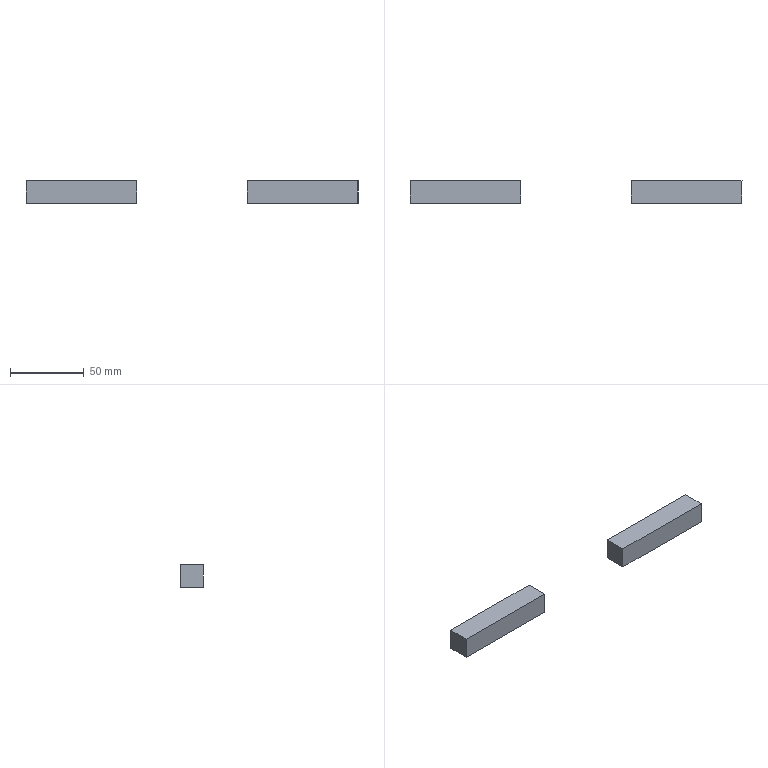Component | SolidWorks | Press-inFixture1-1 | 2 solids | 28 faces | box 225 x 15 x 15 mm | volume 33345 mm3 | plane 12 | cylinder 8 | cone 8 | commonest cylinder face diameters 3.3 x8
build123d program:
from build123d import *

# Parameters (mm, degrees)
SKETCH1_W             = 75
SKETCH1_H             = 15
BOSS_EXTRUDE1_DEPTH   = 15
M4_TAPPED_HOLE2_D     = 3.3
M4_TAPPED_HOLE2_DEPTH = 11.5
M4_TAPPED_HOLE2_TIP   = 0.9914


with BuildPart() as part:
    # Sketch1 → Boss-Extrude1 (new body)
    with BuildSketch(Plane(origin=(0, 0, 0), x_dir=(1, 0, 0), z_dir=(0, 1, 0))):
        Rectangle(SKETCH1_W, SKETCH1_H)
    extrude(amount=BOSS_EXTRUDE1_DEPTH)

    # M4 Tapped Hole2
    with Locations(Plane(origin=(0, 0, 0), x_dir=(-1, 0, 0), z_dir=(0, -1, 0))):
        with Locations((-22.5, 1.5), (22.5, 1.5)):
            Hole(M4_TAPPED_HOLE2_D / 2, depth=M4_TAPPED_HOLE2_DEPTH)
            with Locations((0, 0, -(M4_TAPPED_HOLE2_DEPTH + M4_TAPPED_HOLE2_TIP / 2))):  # 118° drill point
                Cone(0, M4_TAPPED_HOLE2_D / 2, M4_TAPPED_HOLE2_TIP, mode=Mode.SUBTRACT)


with BuildPart() as body_2:
    # Mirror2: mirrored copy
    add(part.part.mirror(Plane.ZY.offset(-75)))


solid = Compound([part.part, body_2.part])

# Placed as in the assembly
solid = solid.moved(Location((-45, -65.5, 208.602), (180, 0, 0)))
STEP:
#1=COLOUR_RGB('',0.7922,0.8196,0.9333);
#2=FILL_AREA_STYLE_COLOUR('',#1);
#3=FILL_AREA_STYLE('',(#2));
#4=SURFACE_STYLE_FILL_AREA(#3);
#5=SURFACE_SIDE_STYLE('',(#4));
#6=SURFACE_STYLE_USAGE(.BOTH.,#5);
#7=PRESENTATION_STYLE_ASSIGNMENT((#6));
#8=CARTESIAN_POINT('',(-0.8858,-3.031,8.207));
#9=VERTEX_POINT('',#8);
#10=CARTESIAN_POINT('',(-0.8858,-3.031,8.337));
#11=VERTEX_POINT('',#10);
#12=CARTESIAN_POINT('',(-0.8858,-3.031,8.272));
#13=DIRECTION('',(-0.,1.,0.));
#14=DIRECTION('',(0.,0.,1.));
#15=AXIS2_PLACEMENT_3D('',#12,#13,#14);
#16=CIRCLE('',#15,0.06496);
#17=EDGE_CURVE('',#9,#11,#16,.T.);
#18=ORIENTED_EDGE('',*,*,#17,.F.);
#19=CARTESIAN_POINT('',(-0.8858,-2.579,8.207));
#20=VERTEX_POINT('',#19);
#21=CARTESIAN_POINT('',(-0.8858,-2.579,8.207));
#22=DIRECTION('',(-0.,1.,0.));
#23=VECTOR('',#22,39.37);
#24=LINE('',#21,#23);
#25=EDGE_CURVE('',#9,#20,#24,.T.);
#26=ORIENTED_EDGE('',*,*,#25,.T.);
#27=CARTESIAN_POINT('',(-0.8858,-2.579,8.337));
#28=VERTEX_POINT('',#27);
#29=CARTESIAN_POINT('',(-0.8858,-2.579,8.272));
#30=DIRECTION('',(-0.,1.,0.));
#31=DIRECTION('',(0.,0.,1.));
#32=AXIS2_PLACEMENT_3D('',#29,#30,#31);
#33=CIRCLE('',#32,0.06496);
#34=EDGE_CURVE('',#20,#28,#33,.T.);
#35=ORIENTED_EDGE('',*,*,#34,.T.);
#36=CARTESIAN_POINT('',(-0.8858,-2.579,8.337));
#37=DIRECTION('',(-0.,1.,0.));
#38=VECTOR('',#37,39.37);
#39=LINE('',#36,#38);
#40=EDGE_CURVE('',#11,#28,#39,.T.);
#41=ORIENTED_EDGE('',*,*,#40,.F.);
#42=EDGE_LOOP('',(#18,#26,#35,#41));
#43=FACE_OUTER_BOUND('',#42,.T.);
#44=CARTESIAN_POINT('',(-0.8858,-2.579,8.272));
#45=DIRECTION('',(-0.,1.,0.));
#46=DIRECTION('',(0.,0.,1.));
#47=AXIS2_PLACEMENT_3D('',#44,#45,#46);
#48=CYLINDRICAL_SURFACE('',#47,0.06496);
#49=ADVANCED_FACE('',(#43),#48,.F.);
#50=CARTESIAN_POINT('',(-0.8858,-3.071,8.272));
#51=VERTEX_POINT('',#50);
#52=CARTESIAN_POINT('',(-0.8858,-3.031,8.337));
#53=DIRECTION('',(-0.,0.515,0.8572));
#54=VECTOR('',#53,39.37);
#55=LINE('',#52,#54);
#56=EDGE_CURVE('',#51,#11,#55,.T.);
#57=ORIENTED_EDGE('',*,*,#56,.F.);
#58=CARTESIAN_POINT('',(-0.8858,-3.031,8.207));
#59=DIRECTION('',(-0.,0.515,-0.8572));
#60=VECTOR('',#59,39.37);
#61=LINE('',#58,#60);
#62=EDGE_CURVE('',#51,#9,#61,.T.);
#63=ORIENTED_EDGE('',*,*,#62,.T.);
#64=ORIENTED_EDGE('',*,*,#17,.T.);
#65=EDGE_LOOP('',(#57,#63,#64));
#66=FACE_OUTER_BOUND('',#65,.T.);
#67=CARTESIAN_POINT('',(-0.8858,-3.031,8.272));
#68=DIRECTION('',(-0.,1.,0.));
#69=DIRECTION('',(0.,0.,1.));
#70=AXIS2_PLACEMENT_3D('',#67,#68,#69);
#71=CONICAL_SURFACE('',#70,0.06496,1.03);
#72=ADVANCED_FACE('',(#66),#71,.F.);
#73=CARTESIAN_POINT('',(-2.657,-3.031,8.207));
#74=VERTEX_POINT('',#73);
#75=CARTESIAN_POINT('',(-2.657,-3.031,8.337));
#76=VERTEX_POINT('',#75);
#77=CARTESIAN_POINT('',(-2.657,-3.031,8.272));
#78=DIRECTION('',(-0.,1.,0.));
#79=DIRECTION('',(0.,0.,1.));
#80=AXIS2_PLACEMENT_3D('',#77,#78,#79);
#81=CIRCLE('',#80,0.06496);
#82=EDGE_CURVE('',#74,#76,#81,.T.);
#83=ORIENTED_EDGE('',*,*,#82,.F.);
#84=CARTESIAN_POINT('',(-2.657,-2.579,8.207));
#85=VERTEX_POINT('',#84);
#86=CARTESIAN_POINT('',(-2.657,-2.579,8.207));
#87=DIRECTION('',(-0.,1.,0.));
#88=VECTOR('',#87,39.37);
#89=LINE('',#86,#88);
#90=EDGE_CURVE('',#74,#85,#89,.T.);
#91=ORIENTED_EDGE('',*,*,#90,.T.);
#92=CARTESIAN_POINT('',(-2.657,-2.579,8.337));
#93=VERTEX_POINT('',#92);
#94=CARTESIAN_POINT('',(-2.657,-2.579,8.272));
#95=DIRECTION('',(-0.,1.,0.));
#96=DIRECTION('',(0.,0.,1.));
#97=AXIS2_PLACEMENT_3D('',#94,#95,#96);
#98=CIRCLE('',#97,0.06496);
#99=EDGE_CURVE('',#85,#93,#98,.T.);
#100=ORIENTED_EDGE('',*,*,#99,.T.);
#101=CARTESIAN_POINT('',(-2.657,-2.579,8.337));
#102=DIRECTION('',(-0.,1.,0.));
#103=VECTOR('',#102,39.37);
#104=LINE('',#101,#103);
#105=EDGE_CURVE('',#76,#93,#104,.T.);
#106=ORIENTED_EDGE('',*,*,#105,.F.);
#107=EDGE_LOOP('',(#83,#91,#100,#106));
#108=FACE_OUTER_BOUND('',#107,.T.);
#109=CARTESIAN_POINT('',(-2.657,-2.579,8.272));
#110=DIRECTION('',(-0.,1.,0.));
#111=DIRECTION('',(0.,0.,1.));
#112=AXIS2_PLACEMENT_3D('',#109,#110,#111);
#113=CYLINDRICAL_SURFACE('',#112,0.06496);
#114=ADVANCED_FACE('',(#108),#113,.F.);
#115=CARTESIAN_POINT('',(-2.657,-3.071,8.272));
#116=VERTEX_POINT('',#115);
#117=CARTESIAN_POINT('',(-2.657,-3.031,8.337));
#118=DIRECTION('',(-0.,0.515,0.8572));
#119=VECTOR('',#118,39.37);
#120=LINE('',#117,#119);
#121=EDGE_CURVE('',#116,#76,#120,.T.);
#122=ORIENTED_EDGE('',*,*,#121,.F.);
#123=CARTESIAN_POINT('',(-2.657,-3.031,8.207));
#124=DIRECTION('',(-0.,0.515,-0.8572));
#125=VECTOR('',#124,39.37);
#126=LINE('',#123,#125);
#127=EDGE_CURVE('',#116,#74,#126,.T.);
#128=ORIENTED_EDGE('',*,*,#127,.T.);
#129=ORIENTED_EDGE('',*,*,#82,.T.);
#130=EDGE_LOOP('',(#122,#128,#129));
#131=FACE_OUTER_BOUND('',#130,.T.);
#132=CARTESIAN_POINT('',(-2.657,-3.031,8.272));
#133=DIRECTION('',(-0.,1.,0.));
#134=DIRECTION('',(0.,0.,1.));
#135=AXIS2_PLACEMENT_3D('',#132,#133,#134);
#136=CONICAL_SURFACE('',#135,0.06496,1.03);
#137=ADVANCED_FACE('',(#131),#136,.F.);
#138=CARTESIAN_POINT('',(-3.248,-2.579,8.508));
#139=VERTEX_POINT('',#138);
#140=CARTESIAN_POINT('',(-3.248,-2.579,7.917));
#141=VERTEX_POINT('',#140);
#142=CARTESIAN_POINT('',(-3.248,-2.579,7.917));
#143=DIRECTION('',(-0.,0.,-1.));
#144=VECTOR('',#143,39.37);
#145=LINE('',#142,#144);
#146=EDGE_CURVE('',#139,#141,#145,.T.);
#147=ORIENTED_EDGE('',*,*,#146,.T.);
#148=CARTESIAN_POINT('',(-3.248,-3.169,7.917));
#149=VERTEX_POINT('',#148);
#150=CARTESIAN_POINT('',(-3.248,-3.169,7.917));
#151=DIRECTION('',(-0.,1.,0.));
#152=VECTOR('',#151,39.37);
#153=LINE('',#150,#152);
#154=EDGE_CURVE('',#149,#141,#153,.T.);
#155=ORIENTED_EDGE('',*,*,#154,.F.);
#156=CARTESIAN_POINT('',(-3.248,-3.169,8.508));
#157=VERTEX_POINT('',#156);
#158=CARTESIAN_POINT('',(-3.248,-3.169,7.917));
#159=DIRECTION('',(-0.,0.,-1.));
#160=VECTOR('',#159,39.37);
#161=LINE('',#158,#160);
#162=EDGE_CURVE('',#157,#149,#161,.T.);
#163=ORIENTED_EDGE('',*,*,#162,.F.);
#164=CARTESIAN_POINT('',(-3.248,-3.169,8.508));
#165=DIRECTION('',(-0.,1.,0.));
#166=VECTOR('',#165,39.37);
#167=LINE('',#164,#166);
#168=EDGE_CURVE('',#157,#139,#167,.T.);
#169=ORIENTED_EDGE('',*,*,#168,.T.);
#170=EDGE_LOOP('',(#147,#155,#163,#169));
#171=FACE_OUTER_BOUND('',#170,.T.);
#172=CARTESIAN_POINT('',(-3.248,-3.169,7.917));
#173=DIRECTION('',(1.,0.,-0.));
#174=DIRECTION('',(0.,-0.,1.));
#175=AXIS2_PLACEMENT_3D('',#172,#173,#174);
#176=PLANE('',#175);
#177=ADVANCED_FACE('',(#171),#176,.F.);
#178=CARTESIAN_POINT('',(-0.2953,-2.579,7.917));
#179=VERTEX_POINT('',#178);
#180=CARTESIAN_POINT('',(-0.2953,-2.579,7.917));
#181=DIRECTION('',(1.,0.,0.));
#182=VECTOR('',#181,39.37);
#183=LINE('',#180,#182);
#184=EDGE_CURVE('',#141,#179,#183,.T.);
#185=ORIENTED_EDGE('',*,*,#184,.T.);
#186=CARTESIAN_POINT('',(-0.2953,-3.169,7.917));
#187=VERTEX_POINT('',#186);
#188=CARTESIAN_POINT('',(-0.2953,-3.169,7.917));
#189=DIRECTION('',(-0.,1.,0.));
#190=VECTOR('',#189,39.37);
#191=LINE('',#188,#190);
#192=EDGE_CURVE('',#187,#179,#191,.T.);
#193=ORIENTED_EDGE('',*,*,#192,.F.);
#194=CARTESIAN_POINT('',(-0.2953,-3.169,7.917));
#195=DIRECTION('',(1.,0.,0.));
#196=VECTOR('',#195,39.37);
#197=LINE('',#194,#196);
#198=EDGE_CURVE('',#149,#187,#197,.T.);
#199=ORIENTED_EDGE('',*,*,#198,.F.);
#200=ORIENTED_EDGE('',*,*,#154,.T.);
#201=EDGE_LOOP('',(#185,#193,#199,#200));
#202=FACE_OUTER_BOUND('',#201,.T.);
#203=CARTESIAN_POINT('',(-0.2953,-3.169,7.917));
#204=DIRECTION('',(-0.,-0.,1.));
#205=DIRECTION('',(-1.,-0.,-0.));
#206=AXIS2_PLACEMENT_3D('',#203,#204,#205);
#207=PLANE('',#206);
#208=ADVANCED_FACE('',(#202),#207,.F.);
#209=CARTESIAN_POINT('',(-0.2953,-2.579,8.508));
#210=VERTEX_POINT('',#209);
#211=CARTESIAN_POINT('',(-0.2953,-2.579,7.917));
#212=DIRECTION('',(0.,-0.,1.));
#213=VECTOR('',#212,39.37);
#214=LINE('',#211,#213);
#215=EDGE_CURVE('',#179,#210,#214,.T.);
#216=ORIENTED_EDGE('',*,*,#215,.T.);
#217=CARTESIAN_POINT('',(-0.2953,-3.169,8.508));
#218=VERTEX_POINT('',#217);
#219=CARTESIAN_POINT('',(-0.2953,-3.169,8.508));
#220=DIRECTION('',(-0.,1.,0.));
#221=VECTOR('',#220,39.37);
#222=LINE('',#219,#221);
#223=EDGE_CURVE('',#218,#210,#222,.T.);
#224=ORIENTED_EDGE('',*,*,#223,.F.);
#225=CARTESIAN_POINT('',(-0.2953,-3.169,7.917));
#226=DIRECTION('',(0.,-0.,1.));
#227=VECTOR('',#226,39.37);
#228=LINE('',#225,#227);
#229=EDGE_CURVE('',#187,#218,#228,.T.);
#230=ORIENTED_EDGE('',*,*,#229,.F.);
#231=ORIENTED_EDGE('',*,*,#192,.T.);
#232=EDGE_LOOP('',(#216,#224,#230,#231));
#233=FACE_OUTER_BOUND('',#232,.T.);
#234=CARTESIAN_POINT('',(-0.2953,-3.169,7.917));
#235=DIRECTION('',(-1.,-0.,0.));
#236=DIRECTION('',(-0.,0.,-1.));
#237=AXIS2_PLACEMENT_3D('',#234,#235,#236);
#238=PLANE('',#237);
#239=ADVANCED_FACE('',(#233),#238,.F.);
#240=CARTESIAN_POINT('',(-0.2953,-2.579,8.508));
#241=DIRECTION('',(-1.,-0.,-0.));
#242=VECTOR('',#241,39.37);
#243=LINE('',#240,#242);
#244=EDGE_CURVE('',#210,#139,#243,.T.);
#245=ORIENTED_EDGE('',*,*,#244,.T.);
#246=ORIENTED_EDGE('',*,*,#168,.F.);
#247=CARTESIAN_POINT('',(-0.2953,-3.169,8.508));
#248=DIRECTION('',(-1.,-0.,-0.));
#249=VECTOR('',#248,39.37);
#250=LINE('',#247,#249);
#251=EDGE_CURVE('',#218,#157,#250,.T.);
#252=ORIENTED_EDGE('',*,*,#251,.F.);
#253=ORIENTED_EDGE('',*,*,#223,.T.);
#254=EDGE_LOOP('',(#245,#246,#252,#253));
#255=FACE_OUTER_BOUND('',#254,.T.);
#256=CARTESIAN_POINT('',(-0.2953,-3.169,8.508));
#257=DIRECTION('',(0.,0.,-1.));
#258=DIRECTION('',(1.,0.,0.));
#259=AXIS2_PLACEMENT_3D('',#256,#257,#258);
#260=PLANE('',#259);
#261=ADVANCED_FACE('',(#255),#260,.F.);
#262=ORIENTED_EDGE('',*,*,#162,.T.);
#263=ORIENTED_EDGE('',*,*,#198,.T.);
#264=ORIENTED_EDGE('',*,*,#229,.T.);
#265=ORIENTED_EDGE('',*,*,#251,.T.);
#266=EDGE_LOOP('',(#262,#263,#264,#265));
#267=FACE_OUTER_BOUND('',#266,.T.);
#268=CARTESIAN_POINT('',(-1.772,-3.169,8.213));
#269=DIRECTION('',(0.,-1.,-0.));
#270=DIRECTION('',(-0.,0.,-1.));
#271=AXIS2_PLACEMENT_3D('',#268,#269,#270);
#272=PLANE('',#271);
#273=ADVANCED_FACE('',(#267),#272,.T.);
#274=CARTESIAN_POINT('',(-0.8858,-2.579,8.272));
#275=DIRECTION('',(-0.,1.,0.));
#276=DIRECTION('',(0.,0.,1.));
#277=AXIS2_PLACEMENT_3D('',#274,#275,#276);
#278=CIRCLE('',#277,0.06496);
#279=EDGE_CURVE('',#28,#20,#278,.T.);
#280=ORIENTED_EDGE('',*,*,#279,.F.);
#281=ORIENTED_EDGE('',*,*,#34,.F.);
#282=EDGE_LOOP('',(#280,#281));
#283=FACE_BOUND('',#282,.T.);
#284=CARTESIAN_POINT('',(-2.657,-2.579,8.272));
#285=DIRECTION('',(-0.,1.,0.));
#286=DIRECTION('',(0.,0.,1.));
#287=AXIS2_PLACEMENT_3D('',#284,#285,#286);
#288=CIRCLE('',#287,0.06496);
#289=EDGE_CURVE('',#93,#85,#288,.T.);
#290=ORIENTED_EDGE('',*,*,#289,.F.);
#291=ORIENTED_EDGE('',*,*,#99,.F.);
#292=EDGE_LOOP('',(#290,#291));
#293=FACE_BOUND('',#292,.T.);
#294=ORIENTED_EDGE('',*,*,#146,.F.);
#295=ORIENTED_EDGE('',*,*,#244,.F.);
#296=ORIENTED_EDGE('',*,*,#215,.F.);
#297=ORIENTED_EDGE('',*,*,#184,.F.);
#298=EDGE_LOOP('',(#294,#295,#296,#297));
#299=FACE_OUTER_BOUND('',#298,.T.);
#300=CARTESIAN_POINT('',(-1.772,-2.579,8.213));
#301=DIRECTION('',(0.,-1.,-0.));
#302=DIRECTION('',(-0.,0.,-1.));
#303=AXIS2_PLACEMENT_3D('',#300,#301,#302);
#304=PLANE('',#303);
#305=ADVANCED_FACE('',(#283,#293,#299),#304,.F.);
#306=ORIENTED_EDGE('',*,*,#127,.F.);
#307=ORIENTED_EDGE('',*,*,#121,.T.);
#308=CARTESIAN_POINT('',(-2.657,-3.031,8.272));
#309=DIRECTION('',(-0.,1.,0.));
#310=DIRECTION('',(0.,0.,1.));
#311=AXIS2_PLACEMENT_3D('',#308,#309,#310);
#312=CIRCLE('',#311,0.06496);
#313=EDGE_CURVE('',#76,#74,#312,.T.);
#314=ORIENTED_EDGE('',*,*,#313,.T.);
#315=EDGE_LOOP('',(#306,#307,#314));
#316=FACE_OUTER_BOUND('',#315,.T.);
#317=CARTESIAN_POINT('',(-2.657,-3.031,8.272));
#318=DIRECTION('',(-0.,1.,0.));
#319=DIRECTION('',(0.,0.,1.));
#320=AXIS2_PLACEMENT_3D('',#317,#318,#319);
#321=CONICAL_SURFACE('',#320,0.06496,1.03);
#322=ADVANCED_FACE('',(#316),#321,.F.);
#323=ORIENTED_EDGE('',*,*,#90,.F.);
#324=ORIENTED_EDGE('',*,*,#313,.F.);
#325=ORIENTED_EDGE('',*,*,#105,.T.);
#326=ORIENTED_EDGE('',*,*,#289,.T.);
#327=EDGE_LOOP('',(#323,#324,#325,#326));
#328=FACE_OUTER_BOUND('',#327,.T.);
#329=CARTESIAN_POINT('',(-2.657,-2.579,8.272));
#330=DIRECTION('',(-0.,1.,0.));
#331=DIRECTION('',(0.,0.,1.));
#332=AXIS2_PLACEMENT_3D('',#329,#330,#331);
#333=CYLINDRICAL_SURFACE('',#332,0.06496);
#334=ADVANCED_FACE('',(#328),#333,.F.);
#335=ORIENTED_EDGE('',*,*,#62,.F.);
#336=ORIENTED_EDGE('',*,*,#56,.T.);
#337=CARTESIAN_POINT('',(-0.8858,-3.031,8.272));
#338=DIRECTION('',(-0.,1.,0.));
#339=DIRECTION('',(0.,0.,1.));
#340=AXIS2_PLACEMENT_3D('',#337,#338,#339);
#341=CIRCLE('',#340,0.06496);
#342=EDGE_CURVE('',#11,#9,#341,.T.);
#343=ORIENTED_EDGE('',*,*,#342,.T.);
#344=EDGE_LOOP('',(#335,#336,#343));
#345=FACE_OUTER_BOUND('',#344,.T.);
#346=CARTESIAN_POINT('',(-0.8858,-3.031,8.272));
#347=DIRECTION('',(-0.,1.,0.));
#348=DIRECTION('',(0.,0.,1.));
#349=AXIS2_PLACEMENT_3D('',#346,#347,#348);
#350=CONICAL_SURFACE('',#349,0.06496,1.03);
#351=ADVANCED_FACE('',(#345),#350,.F.);
#352=ORIENTED_EDGE('',*,*,#25,.F.);
#353=ORIENTED_EDGE('',*,*,#342,.F.);
#354=ORIENTED_EDGE('',*,*,#40,.T.);
#355=ORIENTED_EDGE('',*,*,#279,.T.);
#356=EDGE_LOOP('',(#352,#353,#354,#355));
#357=FACE_OUTER_BOUND('',#356,.T.);
#358=CARTESIAN_POINT('',(-0.8858,-2.579,8.272));
#359=DIRECTION('',(-0.,1.,0.));
#360=DIRECTION('',(0.,0.,1.));
#361=AXIS2_PLACEMENT_3D('',#358,#359,#360);
#362=CYLINDRICAL_SURFACE('',#361,0.06496);
#363=ADVANCED_FACE('',(#357),#362,.F.);
#364=CLOSED_SHELL('',(#49,#72,#114,#137,#177,#208,#239,#261,#273,#305,#322,#334,#351,#363));
#365=MANIFOLD_SOLID_BREP('',#364);
#366=STYLED_ITEM('',(#7),#365);
#367=PRESENTATION_LAYER_ASSIGNMENT('','',(#366));
#368=(LENGTH_UNIT()NAMED_UNIT(*)SI_UNIT($,.METRE.));
#369=LENGTH_MEASURE_WITH_UNIT(LENGTH_MEASURE(0.0254),#368);
#370=DIMENSIONAL_EXPONENTS(1.,0.,0.,0.,0.,0.,0.);
#371=(CONVERSION_BASED_UNIT('',#369)LENGTH_UNIT()NAMED_UNIT(#370));
#372=UNCERTAINTY_MEASURE_WITH_UNIT(LENGTH_MEASURE(0.00001),#371,'','');
#373=(NAMED_UNIT(*)PLANE_ANGLE_UNIT()SI_UNIT($,.RADIAN.));
#374=(NAMED_UNIT(*)SI_UNIT($,.STERADIAN.)SOLID_ANGLE_UNIT());
#375=(GEOMETRIC_REPRESENTATION_CONTEXT(3)GLOBAL_UNCERTAINTY_ASSIGNED_CONTEXT((#372))GLOBAL_UNIT_ASSIGNED_CONTEXT((#371,#373,#374))REPRESENTATION_CONTEXT('',''));
#376=MECHANICAL_DESIGN_GEOMETRIC_PRESENTATION_REPRESENTATION('',(#366),#375);
#377=CARTESIAN_POINT('',(3.248,-3.031,8.337));
#378=VERTEX_POINT('',#377);
#379=CARTESIAN_POINT('',(3.248,-3.031,8.207));
#380=VERTEX_POINT('',#379);
#381=CARTESIAN_POINT('',(3.248,-3.031,8.272));
#382=DIRECTION('',(-0.,-1.,-0.));
#383=DIRECTION('',(0.,0.,1.));
#384=AXIS2_PLACEMENT_3D('',#381,#382,#383);
#385=CIRCLE('',#384,0.06496);
#386=EDGE_CURVE('',#378,#380,#385,.T.);
#387=ORIENTED_EDGE('',*,*,#386,.T.);
#388=CARTESIAN_POINT('',(3.248,-2.579,8.207));
#389=VERTEX_POINT('',#388);
#390=CARTESIAN_POINT('',(3.248,-2.579,8.207));
#391=DIRECTION('',(0.,1.,0.));
#392=VECTOR('',#391,39.37);
#393=LINE('',#390,#392);
#394=EDGE_CURVE('',#380,#389,#393,.T.);
#395=ORIENTED_EDGE('',*,*,#394,.T.);
#396=CARTESIAN_POINT('',(3.248,-2.579,8.337));
#397=VERTEX_POINT('',#396);
#398=CARTESIAN_POINT('',(3.248,-2.579,8.272));
#399=DIRECTION('',(-0.,-1.,-0.));
#400=DIRECTION('',(0.,0.,1.));
#401=AXIS2_PLACEMENT_3D('',#398,#399,#400);
#402=CIRCLE('',#401,0.06496);
#403=EDGE_CURVE('',#397,#389,#402,.T.);
#404=ORIENTED_EDGE('',*,*,#403,.F.);
#405=CARTESIAN_POINT('',(3.248,-2.579,8.337));
#406=DIRECTION('',(0.,1.,0.));
#407=VECTOR('',#406,39.37);
#408=LINE('',#405,#407);
#409=EDGE_CURVE('',#378,#397,#408,.T.);
#410=ORIENTED_EDGE('',*,*,#409,.F.);
#411=EDGE_LOOP('',(#387,#395,#404,#410));
#412=FACE_OUTER_BOUND('',#411,.T.);
#413=CARTESIAN_POINT('',(3.248,-2.579,8.272));
#414=DIRECTION('',(0.,1.,0.));
#415=DIRECTION('',(0.,0.,1.));
#416=AXIS2_PLACEMENT_3D('',#413,#414,#415);
#417=CYLINDRICAL_SURFACE('',#416,0.06496);
#418=ADVANCED_FACE('',(#412),#417,.F.);
#419=CARTESIAN_POINT('',(3.248,-3.071,8.272));
#420=VERTEX_POINT('',#419);
#421=CARTESIAN_POINT('',(3.248,-3.031,8.337));
#422=DIRECTION('',(0.,0.515,0.8572));
#423=VECTOR('',#422,39.37);
#424=LINE('',#421,#423);
#425=EDGE_CURVE('',#420,#378,#424,.T.);
#426=ORIENTED_EDGE('',*,*,#425,.F.);
#427=CARTESIAN_POINT('',(3.248,-3.031,8.207));
#428=DIRECTION('',(0.,0.515,-0.8572));
#429=VECTOR('',#428,39.37);
#430=LINE('',#427,#429);
#431=EDGE_CURVE('',#420,#380,#430,.T.);
#432=ORIENTED_EDGE('',*,*,#431,.T.);
#433=ORIENTED_EDGE('',*,*,#386,.F.);
#434=EDGE_LOOP('',(#426,#432,#433));
#435=FACE_OUTER_BOUND('',#434,.T.);
#436=CARTESIAN_POINT('',(3.248,-3.031,8.272));
#437=DIRECTION('',(0.,1.,0.));
#438=DIRECTION('',(0.,0.,1.));
#439=AXIS2_PLACEMENT_3D('',#436,#437,#438);
#440=CONICAL_SURFACE('',#439,0.06496,1.03);
#441=ADVANCED_FACE('',(#435),#440,.F.);
#442=CARTESIAN_POINT('',(5.02,-3.031,8.337));
#443=VERTEX_POINT('',#442);
#444=CARTESIAN_POINT('',(5.02,-3.031,8.207));
#445=VERTEX_POINT('',#444);
#446=CARTESIAN_POINT('',(5.02,-3.031,8.272));
#447=DIRECTION('',(-0.,-1.,-0.));
#448=DIRECTION('',(0.,0.,1.));
#449=AXIS2_PLACEMENT_3D('',#446,#447,#448);
#450=CIRCLE('',#449,0.06496);
#451=EDGE_CURVE('',#443,#445,#450,.T.);
#452=ORIENTED_EDGE('',*,*,#451,.T.);
#453=CARTESIAN_POINT('',(5.02,-2.579,8.207));
#454=VERTEX_POINT('',#453);
#455=CARTESIAN_POINT('',(5.02,-2.579,8.207));
#456=DIRECTION('',(0.,1.,0.));
#457=VECTOR('',#456,39.37);
#458=LINE('',#455,#457);
#459=EDGE_CURVE('',#445,#454,#458,.T.);
#460=ORIENTED_EDGE('',*,*,#459,.T.);
#461=CARTESIAN_POINT('',(5.02,-2.579,8.337));
#462=VERTEX_POINT('',#461);
#463=CARTESIAN_POINT('',(5.02,-2.579,8.272));
#464=DIRECTION('',(-0.,-1.,-0.));
#465=DIRECTION('',(0.,0.,1.));
#466=AXIS2_PLACEMENT_3D('',#463,#464,#465);
#467=CIRCLE('',#466,0.06496);
#468=EDGE_CURVE('',#462,#454,#467,.T.);
#469=ORIENTED_EDGE('',*,*,#468,.F.);
#470=CARTESIAN_POINT('',(5.02,-2.579,8.337));
#471=DIRECTION('',(0.,1.,0.));
#472=VECTOR('',#471,39.37);
#473=LINE('',#470,#472);
#474=EDGE_CURVE('',#443,#462,#473,.T.);
#475=ORIENTED_EDGE('',*,*,#474,.F.);
#476=EDGE_LOOP('',(#452,#460,#469,#475));
#477=FACE_OUTER_BOUND('',#476,.T.);
#478=CARTESIAN_POINT('',(5.02,-2.579,8.272));
#479=DIRECTION('',(0.,1.,0.));
#480=DIRECTION('',(0.,0.,1.));
#481=AXIS2_PLACEMENT_3D('',#478,#479,#480);
#482=CYLINDRICAL_SURFACE('',#481,0.06496);
#483=ADVANCED_FACE('',(#477),#482,.F.);
#484=CARTESIAN_POINT('',(5.02,-3.071,8.272));
#485=VERTEX_POINT('',#484);
#486=CARTESIAN_POINT('',(5.02,-3.031,8.337));
#487=DIRECTION('',(0.,0.515,0.8572));
#488=VECTOR('',#487,39.37);
#489=LINE('',#486,#488);
#490=EDGE_CURVE('',#485,#443,#489,.T.);
#491=ORIENTED_EDGE('',*,*,#490,.F.);
#492=CARTESIAN_POINT('',(5.02,-3.031,8.207));
#493=DIRECTION('',(0.,0.515,-0.8572));
#494=VECTOR('',#493,39.37);
#495=LINE('',#492,#494);
#496=EDGE_CURVE('',#485,#445,#495,.T.);
#497=ORIENTED_EDGE('',*,*,#496,.T.);
#498=ORIENTED_EDGE('',*,*,#451,.F.);
#499=EDGE_LOOP('',(#491,#497,#498));
#500=FACE_OUTER_BOUND('',#499,.T.);
#501=CARTESIAN_POINT('',(5.02,-3.031,8.272));
#502=DIRECTION('',(0.,1.,0.));
#503=DIRECTION('',(0.,0.,1.));
#504=AXIS2_PLACEMENT_3D('',#501,#502,#503);
#505=CONICAL_SURFACE('',#504,0.06496,1.03);
#506=ADVANCED_FACE('',(#500),#505,.F.);
#507=CARTESIAN_POINT('',(5.61,-2.579,8.508));
#508=VERTEX_POINT('',#507);
#509=CARTESIAN_POINT('',(5.61,-2.579,7.917));
#510=VERTEX_POINT('',#509);
#511=CARTESIAN_POINT('',(5.61,-2.579,7.917));
#512=DIRECTION('',(0.,0.,-1.));
#513=VECTOR('',#512,39.37);
#514=LINE('',#511,#513);
#515=EDGE_CURVE('',#508,#510,#514,.T.);
#516=ORIENTED_EDGE('',*,*,#515,.F.);
#517=CARTESIAN_POINT('',(5.61,-3.169,8.508));
#518=VERTEX_POINT('',#517);
#519=CARTESIAN_POINT('',(5.61,-3.169,8.508));
#520=DIRECTION('',(0.,1.,0.));
#521=VECTOR('',#520,39.37);
#522=LINE('',#519,#521);
#523=EDGE_CURVE('',#518,#508,#522,.T.);
#524=ORIENTED_EDGE('',*,*,#523,.F.);
#525=CARTESIAN_POINT('',(5.61,-3.169,7.917));
#526=VERTEX_POINT('',#525);
#527=CARTESIAN_POINT('',(5.61,-3.169,7.917));
#528=DIRECTION('',(0.,0.,-1.));
#529=VECTOR('',#528,39.37);
#530=LINE('',#527,#529);
#531=EDGE_CURVE('',#518,#526,#530,.T.);
#532=ORIENTED_EDGE('',*,*,#531,.T.);
#533=CARTESIAN_POINT('',(5.61,-3.169,7.917));
#534=DIRECTION('',(0.,1.,0.));
#535=VECTOR('',#534,39.37);
#536=LINE('',#533,#535);
#537=EDGE_CURVE('',#526,#510,#536,.T.);
#538=ORIENTED_EDGE('',*,*,#537,.T.);
#539=EDGE_LOOP('',(#516,#524,#532,#538));
#540=FACE_OUTER_BOUND('',#539,.T.);
#541=CARTESIAN_POINT('',(5.61,-3.169,7.917));
#542=DIRECTION('',(-1.,0.,-0.));
#543=DIRECTION('',(-0.,-0.,1.));
#544=AXIS2_PLACEMENT_3D('',#541,#542,#543);
#545=PLANE('',#544);
#546=ADVANCED_FACE('',(#540),#545,.F.);
#547=CARTESIAN_POINT('',(2.657,-2.579,7.917));
#548=VERTEX_POINT('',#547);
#549=CARTESIAN_POINT('',(2.657,-2.579,7.917));
#550=DIRECTION('',(-1.,0.,-0.));
#551=VECTOR('',#550,39.37);
#552=LINE('',#549,#551);
#553=EDGE_CURVE('',#510,#548,#552,.T.);
#554=ORIENTED_EDGE('',*,*,#553,.F.);
#555=ORIENTED_EDGE('',*,*,#537,.F.);
#556=CARTESIAN_POINT('',(2.657,-3.169,7.917));
#557=VERTEX_POINT('',#556);
#558=CARTESIAN_POINT('',(2.657,-3.169,7.917));
#559=DIRECTION('',(-1.,0.,-0.));
#560=VECTOR('',#559,39.37);
#561=LINE('',#558,#560);
#562=EDGE_CURVE('',#526,#557,#561,.T.);
#563=ORIENTED_EDGE('',*,*,#562,.T.);
#564=CARTESIAN_POINT('',(2.657,-3.169,7.917));
#565=DIRECTION('',(0.,1.,0.));
#566=VECTOR('',#565,39.37);
#567=LINE('',#564,#566);
#568=EDGE_CURVE('',#557,#548,#567,.T.);
#569=ORIENTED_EDGE('',*,*,#568,.T.);
#570=EDGE_LOOP('',(#554,#555,#563,#569));
#571=FACE_OUTER_BOUND('',#570,.T.);
#572=CARTESIAN_POINT('',(2.657,-3.169,7.917));
#573=DIRECTION('',(-0.,-0.,1.));
#574=DIRECTION('',(1.,-0.,0.));
#575=AXIS2_PLACEMENT_3D('',#572,#573,#574);
#576=PLANE('',#575);
#577=ADVANCED_FACE('',(#571),#576,.F.);
#578=CARTESIAN_POINT('',(2.657,-2.579,8.508));
#579=VERTEX_POINT('',#578);
#580=CARTESIAN_POINT('',(2.657,-2.579,7.917));
#581=DIRECTION('',(-0.,-0.,1.));
#582=VECTOR('',#581,39.37);
#583=LINE('',#580,#582);
#584=EDGE_CURVE('',#548,#579,#583,.T.);
#585=ORIENTED_EDGE('',*,*,#584,.F.);
#586=ORIENTED_EDGE('',*,*,#568,.F.);
#587=CARTESIAN_POINT('',(2.657,-3.169,8.508));
#588=VERTEX_POINT('',#587);
#589=CARTESIAN_POINT('',(2.657,-3.169,7.917));
#590=DIRECTION('',(-0.,-0.,1.));
#591=VECTOR('',#590,39.37);
#592=LINE('',#589,#591);
#593=EDGE_CURVE('',#557,#588,#592,.T.);
#594=ORIENTED_EDGE('',*,*,#593,.T.);
#595=CARTESIAN_POINT('',(2.657,-3.169,8.508));
#596=DIRECTION('',(0.,1.,0.));
#597=VECTOR('',#596,39.37);
#598=LINE('',#595,#597);
#599=EDGE_CURVE('',#588,#579,#598,.T.);
#600=ORIENTED_EDGE('',*,*,#599,.T.);
#601=EDGE_LOOP('',(#585,#586,#594,#600));
#602=FACE_OUTER_BOUND('',#601,.T.);
#603=CARTESIAN_POINT('',(2.657,-3.169,7.917));
#604=DIRECTION('',(1.,-0.,0.));
#605=DIRECTION('',(0.,0.,-1.));
#606=AXIS2_PLACEMENT_3D('',#603,#604,#605);
#607=PLANE('',#606);
#608=ADVANCED_FACE('',(#602),#607,.F.);
#609=CARTESIAN_POINT('',(2.657,-2.579,8.508));
#610=DIRECTION('',(1.,-0.,0.));
#611=VECTOR('',#610,39.37);
#612=LINE('',#609,#611);
#613=EDGE_CURVE('',#579,#508,#612,.T.);
#614=ORIENTED_EDGE('',*,*,#613,.F.);
#615=ORIENTED_EDGE('',*,*,#599,.F.);
#616=CARTESIAN_POINT('',(2.657,-3.169,8.508));
#617=DIRECTION('',(1.,-0.,0.));
#618=VECTOR('',#617,39.37);
#619=LINE('',#616,#618);
#620=EDGE_CURVE('',#588,#518,#619,.T.);
#621=ORIENTED_EDGE('',*,*,#620,.T.);
#622=ORIENTED_EDGE('',*,*,#523,.T.);
#623=EDGE_LOOP('',(#614,#615,#621,#622));
#624=FACE_OUTER_BOUND('',#623,.T.);
#625=CARTESIAN_POINT('',(2.657,-3.169,8.508));
#626=DIRECTION('',(0.,0.,-1.));
#627=DIRECTION('',(-1.,0.,-0.));
#628=AXIS2_PLACEMENT_3D('',#625,#626,#627);
#629=PLANE('',#628);
#630=ADVANCED_FACE('',(#624),#629,.F.);
#631=ORIENTED_EDGE('',*,*,#531,.F.);
#632=ORIENTED_EDGE('',*,*,#620,.F.);
#633=ORIENTED_EDGE('',*,*,#593,.F.);
#634=ORIENTED_EDGE('',*,*,#562,.F.);
#635=EDGE_LOOP('',(#631,#632,#633,#634));
#636=FACE_OUTER_BOUND('',#635,.T.);
#637=CARTESIAN_POINT('',(4.134,-3.169,8.213));
#638=DIRECTION('',(-0.,-1.,-0.));
#639=DIRECTION('',(0.,0.,-1.));
#640=AXIS2_PLACEMENT_3D('',#637,#638,#639);
#641=PLANE('',#640);
#642=ADVANCED_FACE('',(#636),#641,.T.);
#643=ORIENTED_EDGE('',*,*,#403,.T.);
#644=CARTESIAN_POINT('',(3.248,-2.579,8.272));
#645=DIRECTION('',(-0.,-1.,-0.));
#646=DIRECTION('',(0.,0.,1.));
#647=AXIS2_PLACEMENT_3D('',#644,#645,#646);
#648=CIRCLE('',#647,0.06496);
#649=EDGE_CURVE('',#389,#397,#648,.T.);
#650=ORIENTED_EDGE('',*,*,#649,.T.);
#651=EDGE_LOOP('',(#643,#650));
#652=FACE_BOUND('',#651,.T.);
#653=ORIENTED_EDGE('',*,*,#468,.T.);
#654=CARTESIAN_POINT('',(5.02,-2.579,8.272));
#655=DIRECTION('',(-0.,-1.,-0.));
#656=DIRECTION('',(0.,0.,1.));
#657=AXIS2_PLACEMENT_3D('',#654,#655,#656);
#658=CIRCLE('',#657,0.06496);
#659=EDGE_CURVE('',#454,#462,#658,.T.);
#660=ORIENTED_EDGE('',*,*,#659,.T.);
#661=EDGE_LOOP('',(#653,#660));
#662=FACE_BOUND('',#661,.T.);
#663=ORIENTED_EDGE('',*,*,#515,.T.);
#664=ORIENTED_EDGE('',*,*,#553,.T.);
#665=ORIENTED_EDGE('',*,*,#584,.T.);
#666=ORIENTED_EDGE('',*,*,#613,.T.);
#667=EDGE_LOOP('',(#663,#664,#665,#666));
#668=FACE_OUTER_BOUND('',#667,.T.);
#669=CARTESIAN_POINT('',(4.134,-2.579,8.213));
#670=DIRECTION('',(-0.,-1.,-0.));
#671=DIRECTION('',(0.,0.,-1.));
#672=AXIS2_PLACEMENT_3D('',#669,#670,#671);
#673=PLANE('',#672);
#674=ADVANCED_FACE('',(#652,#662,#668),#673,.F.);
#675=ORIENTED_EDGE('',*,*,#496,.F.);
#676=ORIENTED_EDGE('',*,*,#490,.T.);
#677=CARTESIAN_POINT('',(5.02,-3.031,8.272));
#678=DIRECTION('',(-0.,-1.,-0.));
#679=DIRECTION('',(0.,0.,1.));
#680=AXIS2_PLACEMENT_3D('',#677,#678,#679);
#681=CIRCLE('',#680,0.06496);
#682=EDGE_CURVE('',#445,#443,#681,.T.);
#683=ORIENTED_EDGE('',*,*,#682,.F.);
#684=EDGE_LOOP('',(#675,#676,#683));
#685=FACE_OUTER_BOUND('',#684,.T.);
#686=CARTESIAN_POINT('',(5.02,-3.031,8.272));
#687=DIRECTION('',(0.,1.,0.));
#688=DIRECTION('',(0.,0.,1.));
#689=AXIS2_PLACEMENT_3D('',#686,#687,#688);
#690=CONICAL_SURFACE('',#689,0.06496,1.03);
#691=ADVANCED_FACE('',(#685),#690,.F.);
#692=ORIENTED_EDGE('',*,*,#459,.F.);
#693=ORIENTED_EDGE('',*,*,#682,.T.);
#694=ORIENTED_EDGE('',*,*,#474,.T.);
#695=ORIENTED_EDGE('',*,*,#659,.F.);
#696=EDGE_LOOP('',(#692,#693,#694,#695));
#697=FACE_OUTER_BOUND('',#696,.T.);
#698=CARTESIAN_POINT('',(5.02,-2.579,8.272));
#699=DIRECTION('',(0.,1.,0.));
#700=DIRECTION('',(0.,0.,1.));
#701=AXIS2_PLACEMENT_3D('',#698,#699,#700);
#702=CYLINDRICAL_SURFACE('',#701,0.06496);
#703=ADVANCED_FACE('',(#697),#702,.F.);
#704=ORIENTED_EDGE('',*,*,#431,.F.);
#705=ORIENTED_EDGE('',*,*,#425,.T.);
#706=CARTESIAN_POINT('',(3.248,-3.031,8.272));
#707=DIRECTION('',(-0.,-1.,-0.));
#708=DIRECTION('',(0.,0.,1.));
#709=AXIS2_PLACEMENT_3D('',#706,#707,#708);
#710=CIRCLE('',#709,0.06496);
#711=EDGE_CURVE('',#380,#378,#710,.T.);
#712=ORIENTED_EDGE('',*,*,#711,.F.);
#713=EDGE_LOOP('',(#704,#705,#712));
#714=FACE_OUTER_BOUND('',#713,.T.);
#715=CARTESIAN_POINT('',(3.248,-3.031,8.272));
#716=DIRECTION('',(0.,1.,0.));
#717=DIRECTION('',(0.,0.,1.));
#718=AXIS2_PLACEMENT_3D('',#715,#716,#717);
#719=CONICAL_SURFACE('',#718,0.06496,1.03);
#720=ADVANCED_FACE('',(#714),#719,.F.);
#721=ORIENTED_EDGE('',*,*,#394,.F.);
#722=ORIENTED_EDGE('',*,*,#711,.T.);
#723=ORIENTED_EDGE('',*,*,#409,.T.);
#724=ORIENTED_EDGE('',*,*,#649,.F.);
#725=EDGE_LOOP('',(#721,#722,#723,#724));
#726=FACE_OUTER_BOUND('',#725,.T.);
#727=CARTESIAN_POINT('',(3.248,-2.579,8.272));
#728=DIRECTION('',(0.,1.,0.));
#729=DIRECTION('',(0.,0.,1.));
#730=AXIS2_PLACEMENT_3D('',#727,#728,#729);
#731=CYLINDRICAL_SURFACE('',#730,0.06496);
#732=ADVANCED_FACE('',(#726),#731,.F.);
#733=CLOSED_SHELL('',(#418,#441,#483,#506,#546,#577,#608,#630,#642,#674,#691,#703,#720,#732));
#734=MANIFOLD_SOLID_BREP('',#733);
#735=CARTESIAN_POINT('',(0.,0.,0.));
#736=DIRECTION('',(0.,0.,1.));
#737=DIRECTION('',(1.,0.,0.));
#738=AXIS2_PLACEMENT_3D('',#735,#736,#737);
#739=(LENGTH_UNIT()NAMED_UNIT(*)SI_UNIT($,.METRE.));
#740=LENGTH_MEASURE_WITH_UNIT(LENGTH_MEASURE(0.0254),#739);
#741=DIMENSIONAL_EXPONENTS(1.,0.,0.,0.,0.,0.,0.);
#742=(CONVERSION_BASED_UNIT('',#740)LENGTH_UNIT()NAMED_UNIT(#741));
#743=UNCERTAINTY_MEASURE_WITH_UNIT(LENGTH_MEASURE(0.00001),#742,'','');
#744=(NAMED_UNIT(*)PLANE_ANGLE_UNIT()SI_UNIT($,.RADIAN.));
#745=(NAMED_UNIT(*)SI_UNIT($,.STERADIAN.)SOLID_ANGLE_UNIT());
#746=(GEOMETRIC_REPRESENTATION_CONTEXT(3)GLOBAL_UNCERTAINTY_ASSIGNED_CONTEXT((#743))GLOBAL_UNIT_ASSIGNED_CONTEXT((#742,#744,#745))REPRESENTATION_CONTEXT('',''));
#747=ADVANCED_BREP_SHAPE_REPRESENTATION('',(#734,#365,#738),#746);
#748=COLOUR_RGB('',0.7922,0.8196,0.9333);
#749=FILL_AREA_STYLE_COLOUR('',#748);
#750=FILL_AREA_STYLE('',(#749));
#751=SURFACE_STYLE_FILL_AREA(#750);
#752=SURFACE_SIDE_STYLE('',(#751));
#753=SURFACE_STYLE_USAGE(.BOTH.,#752);
#754=PRESENTATION_STYLE_ASSIGNMENT((#753));
#755=STYLED_ITEM('',(#754),#734);
#756=PRESENTATION_LAYER_ASSIGNMENT('','',(#755));
#757=(LENGTH_UNIT()NAMED_UNIT(*)SI_UNIT($,.METRE.));
#758=LENGTH_MEASURE_WITH_UNIT(LENGTH_MEASURE(0.0254),#757);
#759=DIMENSIONAL_EXPONENTS(1.,0.,0.,0.,0.,0.,0.);
#760=(CONVERSION_BASED_UNIT('',#758)LENGTH_UNIT()NAMED_UNIT(#759));
#761=UNCERTAINTY_MEASURE_WITH_UNIT(LENGTH_MEASURE(0.00001),#760,'','');
#762=(NAMED_UNIT(*)PLANE_ANGLE_UNIT()SI_UNIT($,.RADIAN.));
#763=(NAMED_UNIT(*)SI_UNIT($,.STERADIAN.)SOLID_ANGLE_UNIT());
#764=(GEOMETRIC_REPRESENTATION_CONTEXT(3)GLOBAL_UNCERTAINTY_ASSIGNED_CONTEXT((#761))GLOBAL_UNIT_ASSIGNED_CONTEXT((#760,#762,#763))REPRESENTATION_CONTEXT('',''));
#765=MECHANICAL_DESIGN_GEOMETRIC_PRESENTATION_REPRESENTATION('',(#755),#764);